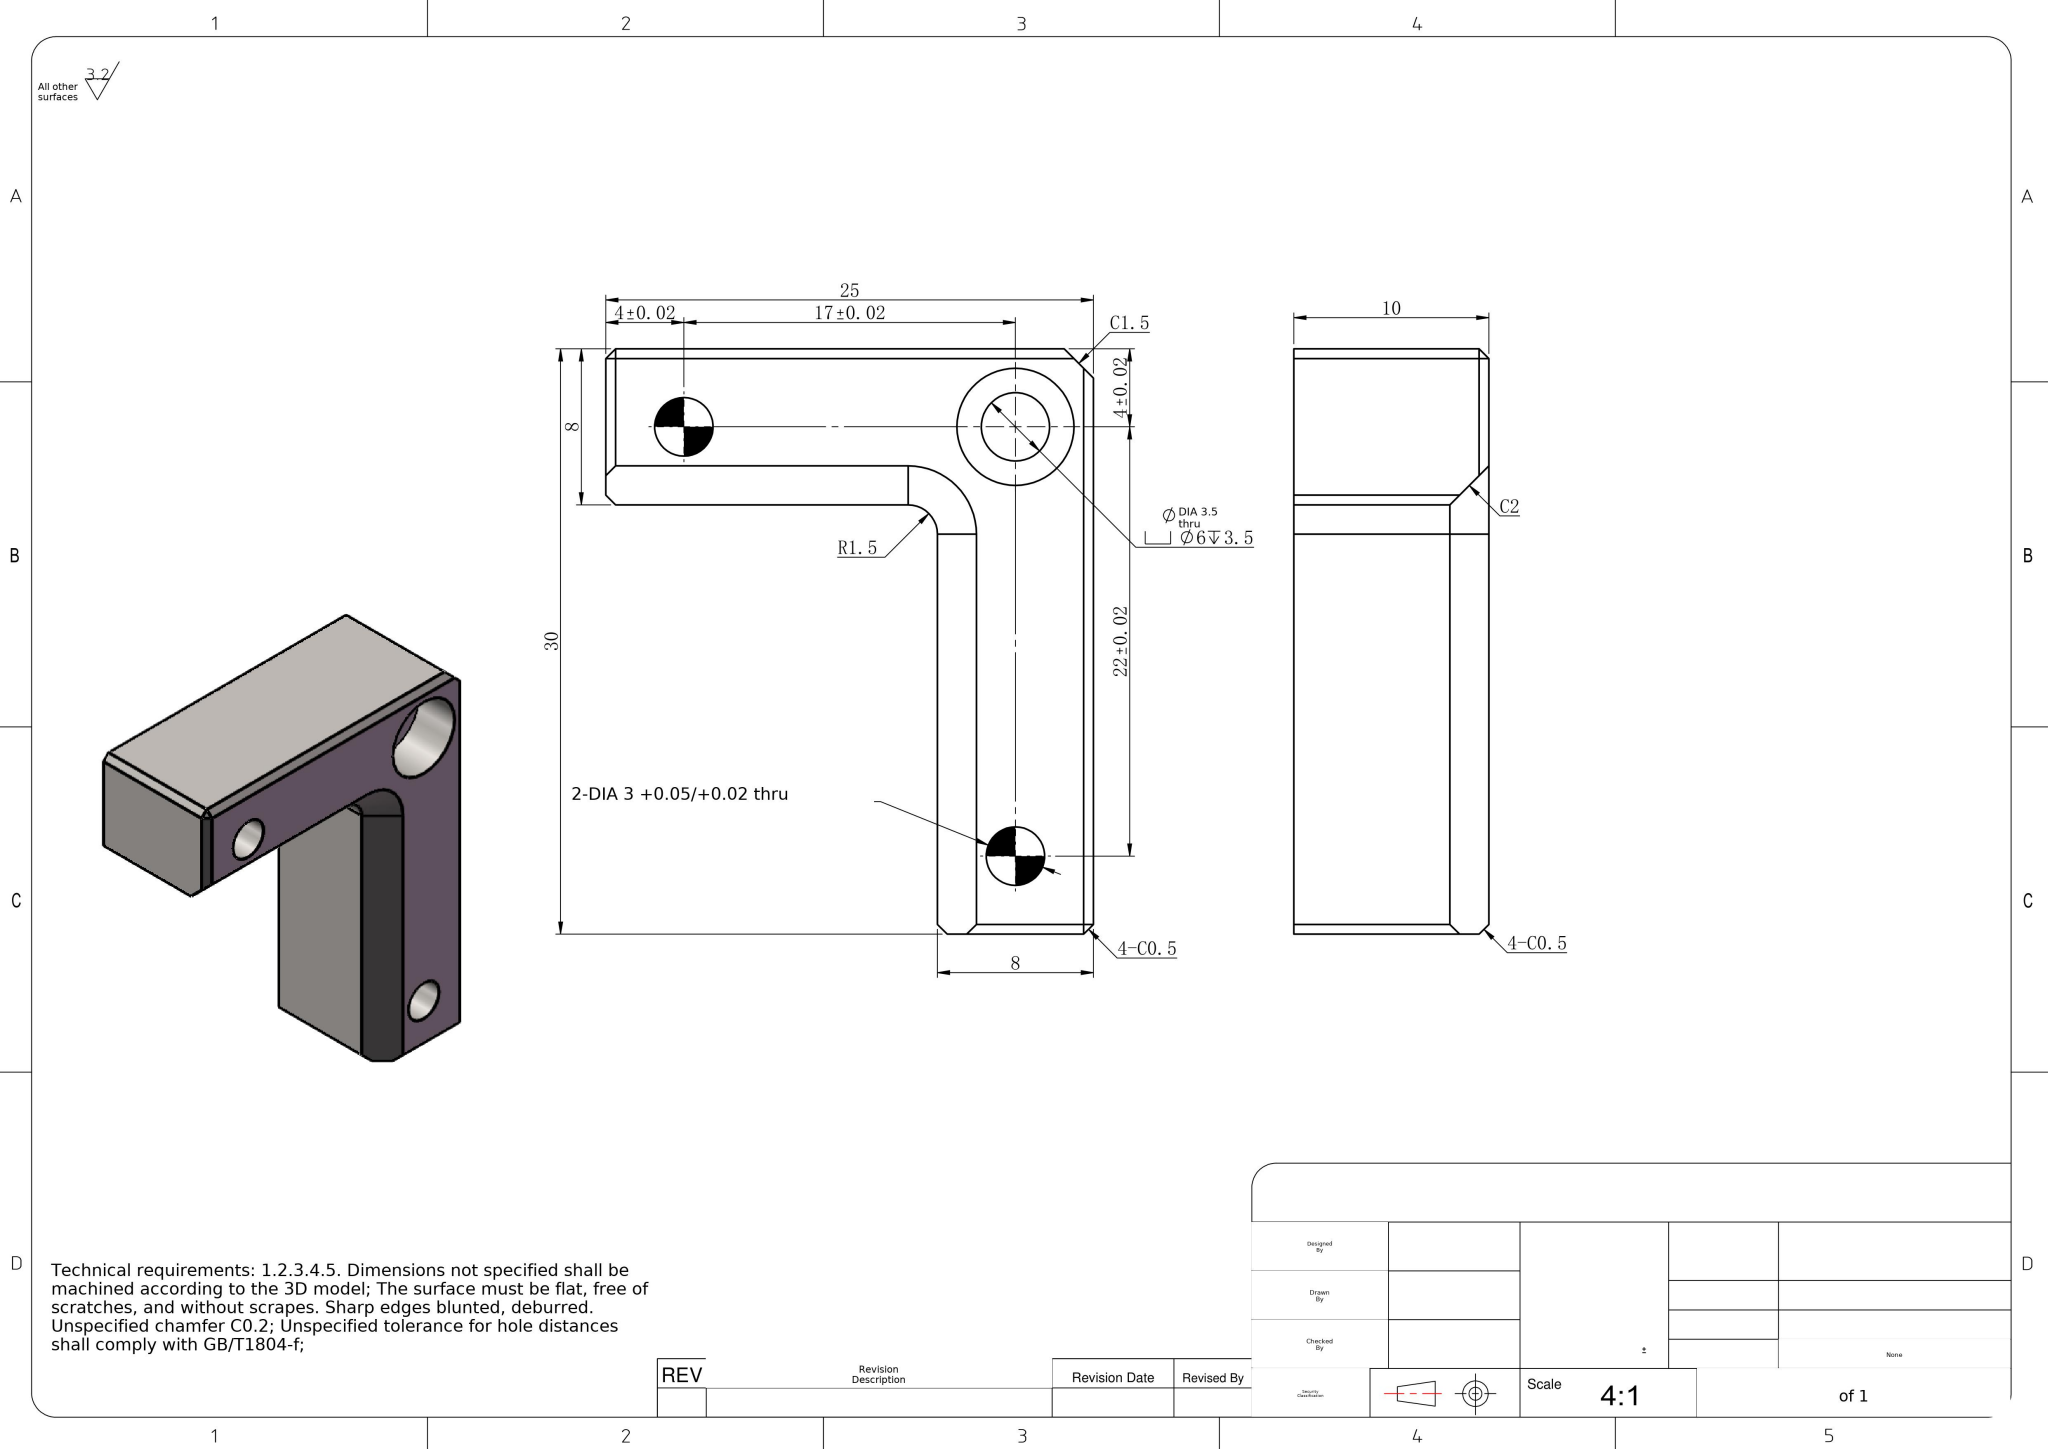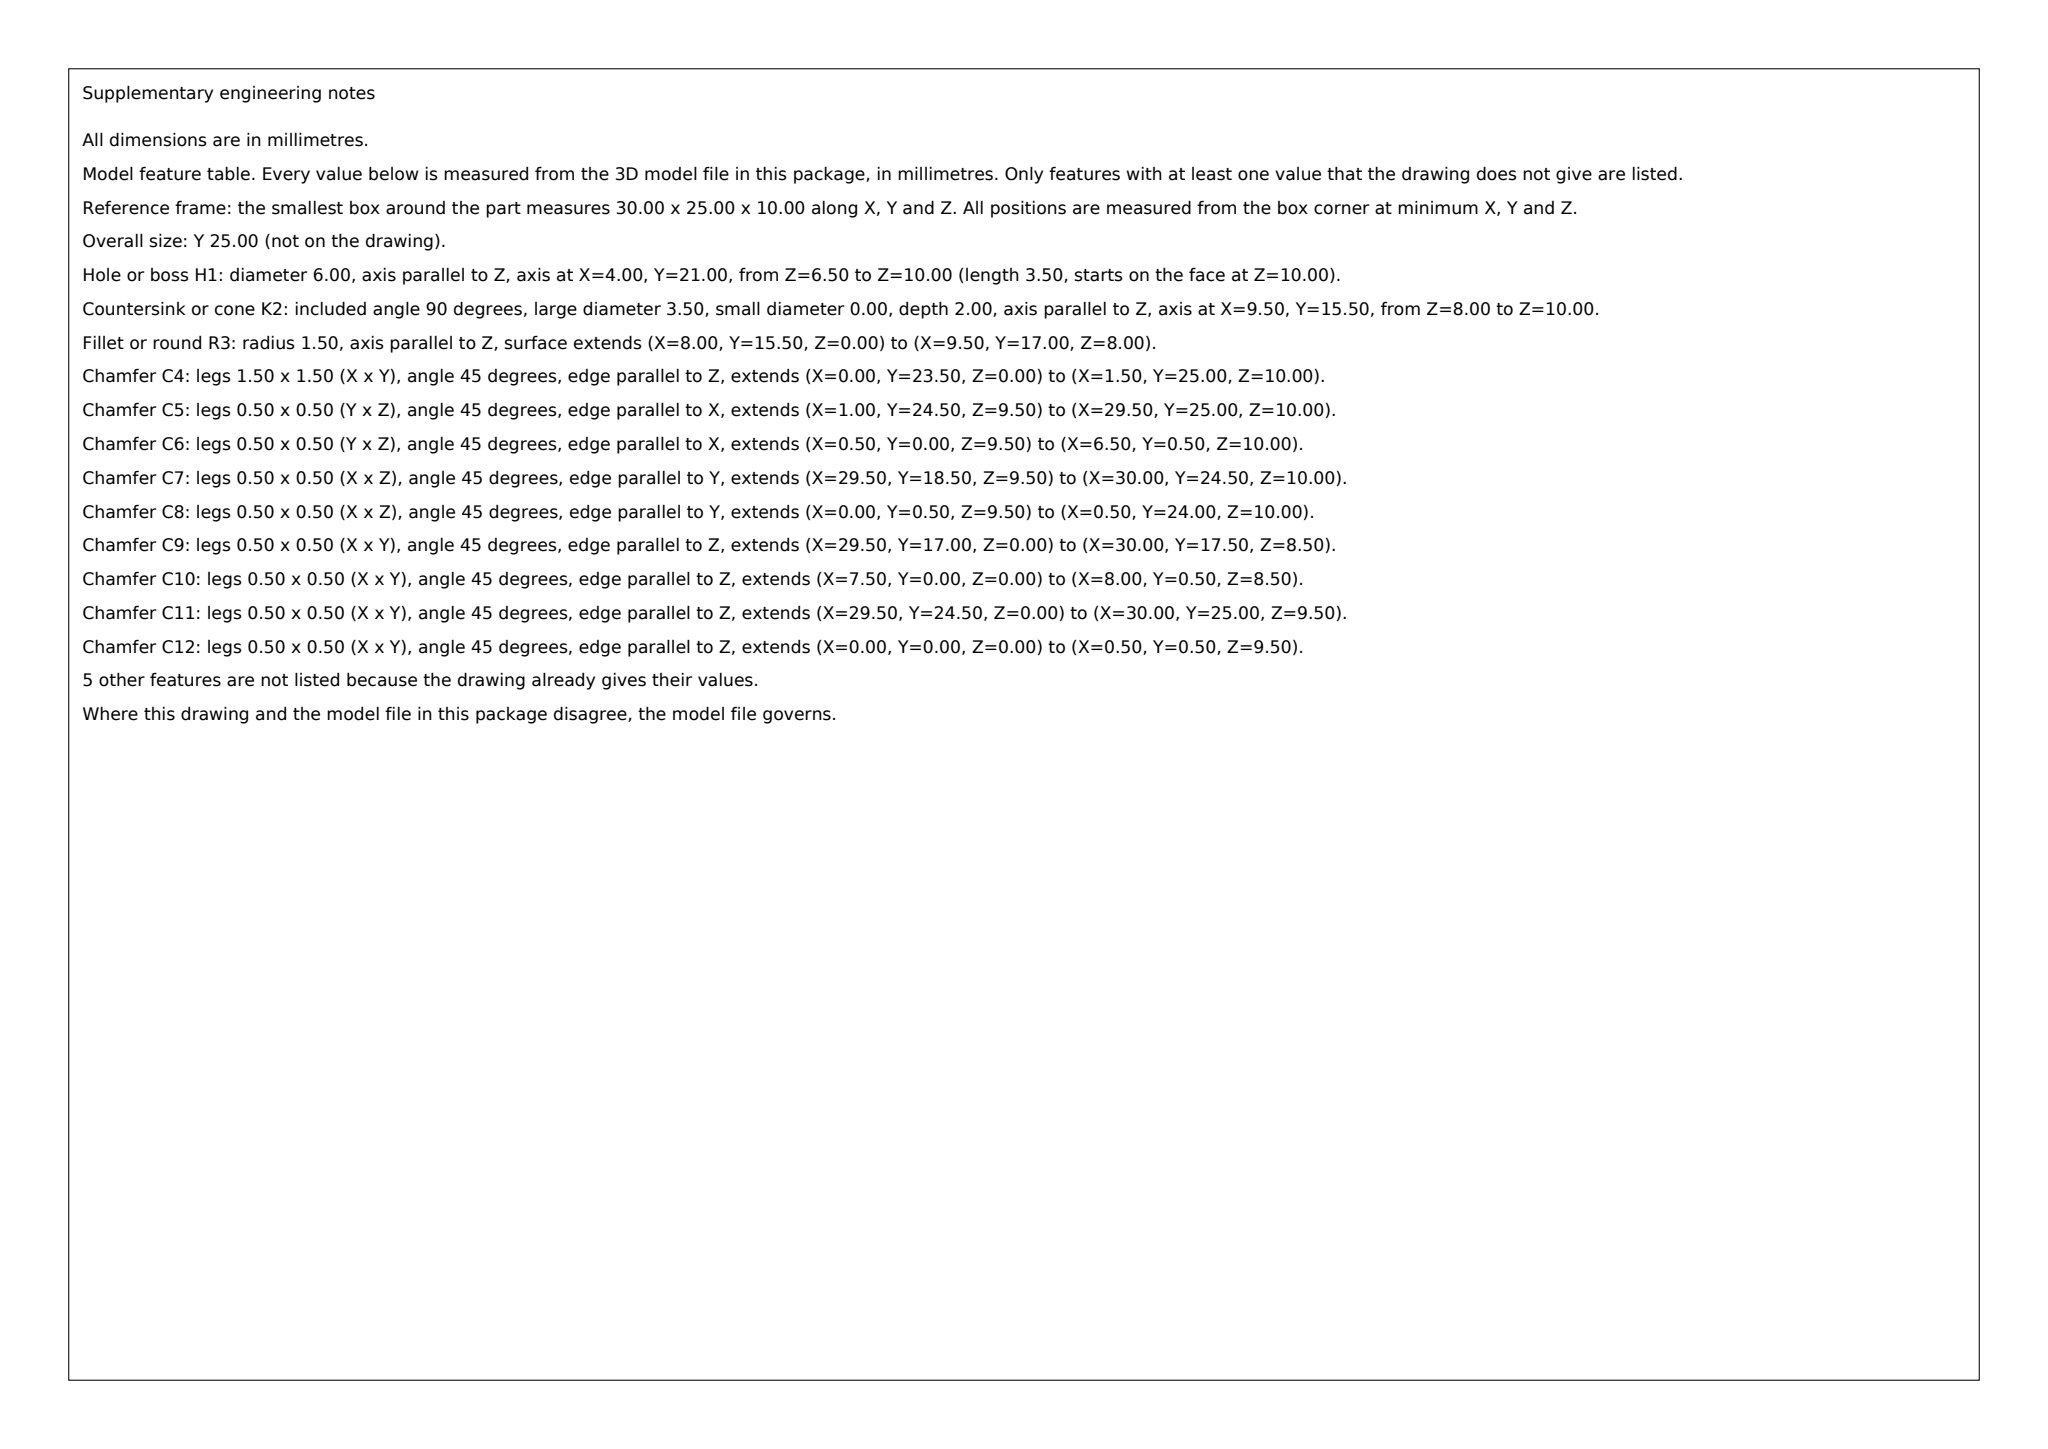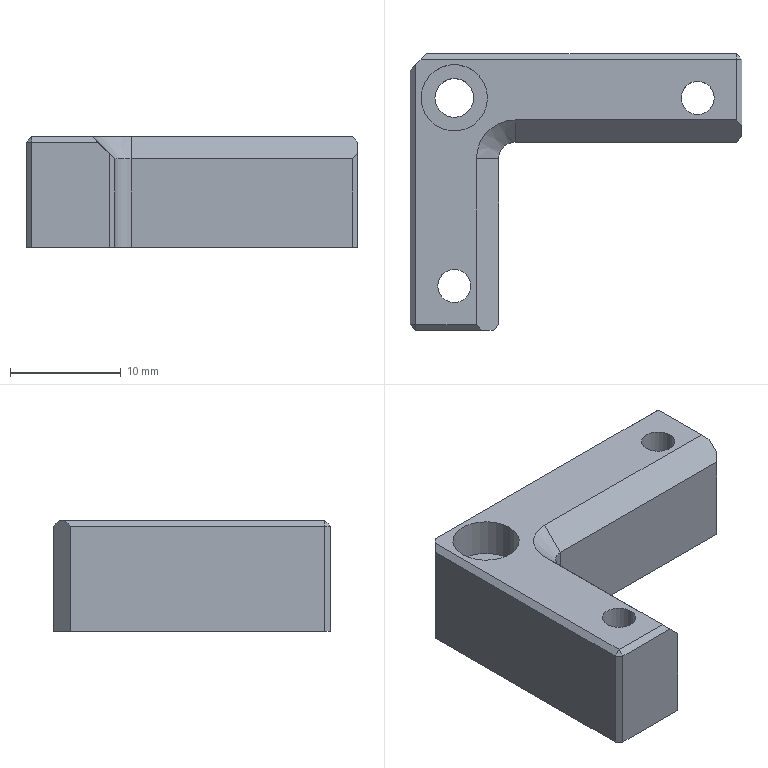Part | SolidWorks | mm | 1 solid | 32 faces | box 30 x 25 x 10 mm | volume 3359 mm3 | plane 22 | cylinder 9 | cone 1 | commonest cylinder face diameters 3 x5 6 x2 3.5 x2
build123d program:
from build123d import *

# Parameters (mm, degrees)
SKETCH1_W                                         = 30
SKETCH1_H                                         = 25
BOSS_EXTRUDE1_DEPTH                               = 10
SKETCH2_W                                         = 22
SKETCH2_H                                         = 17
CUT_EXTRUDE1_DEPTH                                = 22.937
FILLET1_R                                         = 1.5
CHAMFER1_SIZE                                     = 2
HOLE_SIZE_ACCORDING_TO_SLOTTED_PAN_HE_D           = 3.5
HOLE_SIZE_ACCORDING_TO_SLOTTED_PAN_HE_CBORE_D     = 6
HOLE_SIZE_ACCORDING_TO_SLOTTED_PAN_HE_CBORE_DEPTH = 3.5
SKETCH5_R                                         = 1.5
CUT_EXTRUDE2_DEPTH                                = 22.937
CHAMFER2_SIZE                                     = 1.5
CHAMFER3_SIZE                                     = 0.5


with BuildPart() as part:
    # Sketch1 → Boss-Extrude1 (new body)
    with BuildSketch(Plane.XY):
        Rectangle(SKETCH1_W, SKETCH1_H)
    extrude(amount=BOSS_EXTRUDE1_DEPTH)

    # Sketch2 → Cut-Extrude1 (cut, through all)
    with BuildSketch(Plane.XY.offset(10)):
        with Locations((4, -4)):
            Rectangle(SKETCH2_W, SKETCH2_H)
    extrude(amount=-CUT_EXTRUDE1_DEPTH, mode=Mode.SUBTRACT)

    # Fillet1
    fillet1_edges = [part.edges().sort_by_distance(p)[0] for p in [
        (-7, 4.5, 5),
    ]]
    fillet(fillet1_edges, radius=FILLET1_R)

    # Chamfer1
    chamfer1_edges = [part.edges().sort_by_distance(p)[0] for p in [
        (4.75, 4.5, 10),
        (-7, -4.75, 10),
        (-6.561, 4.061, 10),
    ]]
    chamfer(chamfer1_edges, length=CHAMFER1_SIZE)

    # Hole Size _ according to_ Slotted Pan He (through all)
    with Locations(Plane.XY.offset(10)):
        with Locations((-11, 8.5)):
            CounterBoreHole(HOLE_SIZE_ACCORDING_TO_SLOTTED_PAN_HE_D / 2, HOLE_SIZE_ACCORDING_TO_SLOTTED_PAN_HE_CBORE_D / 2, HOLE_SIZE_ACCORDING_TO_SLOTTED_PAN_HE_CBORE_DEPTH)

    # Sketch5 → Cut-Extrude2 (cut, through all)
    with BuildSketch(Plane.XY.offset(10)):
        with Locations((11, 8.5)):
            Circle(SKETCH5_R)
        with Locations((-11, -8.5)):
            Circle(SKETCH5_R)
    extrude(amount=-CUT_EXTRUDE2_DEPTH, mode=Mode.SUBTRACT)

    # Chamfer2
    chamfer2_edges = [part.edges().sort_by_distance(p)[0] for p in [
        (-15, 12.5, 5),
    ]]
    chamfer(chamfer2_edges, length=CHAMFER2_SIZE)

    # Chamfer3
    chamfer3_edges = [part.edges().sort_by_distance(p)[0] for p in [
        (-12, -12.5, 10),
        (15, 4.5, 4),
        (-7, -12.5, 4),
        (15, 9.5, 10),
        (-15, -0.75, 10),
        (0.75, 12.5, 10),
        (-15, -12.5, 5),
        (15, 12.5, 5),
    ]]
    chamfer(chamfer3_edges, length=CHAMFER3_SIZE)


solid = part.part